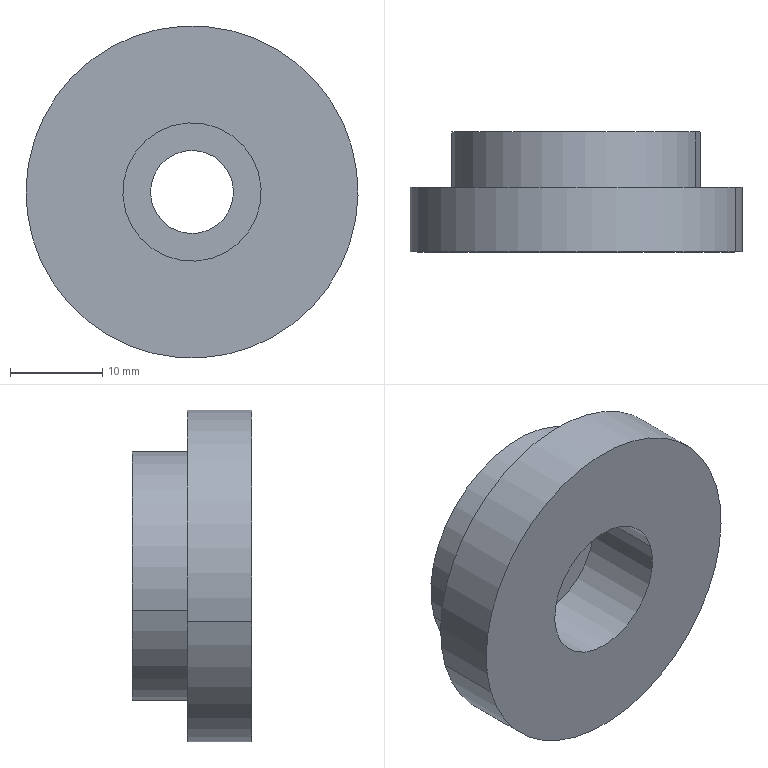Component | SolidWorks | NewDieSet-1_SpacerBlock-1 | 1 solid | 12 faces | box 36 x 13 x 36 mm | volume 8716 mm3 | cylinder 8 | plane 4 | commonest cylinder face diameters 15 x2 9 x2 27 x2 36 x2
build123d program:
from build123d import *

# Parameters (mm, degrees)
SKETCH1_R                                            = 18
BOSS_EXTRUDE1_DEPTH                                  = 7
SKETCH4_R                                            = 13.5
BOSS_EXTRUDE2_DEPTH                                  = 6
HOLE_SIZE_ACCORDING_TO_HEXAGON_SOCKET_HE_D           = 9
HOLE_SIZE_ACCORDING_TO_HEXAGON_SOCKET_HE_CBORE_D     = 15
HOLE_SIZE_ACCORDING_TO_HEXAGON_SOCKET_HE_CBORE_DEPTH = 9


with BuildPart() as part:
    # Sketch1 → Boss-Extrude1 (new body)
    with BuildSketch(Plane.XY):
        Circle(SKETCH1_R)
    extrude(amount=BOSS_EXTRUDE1_DEPTH)

    # Sketch4 → Boss-Extrude2 (add)
    with BuildSketch(Plane(origin=(0, 0, 0), x_dir=(-1, 0, 0), z_dir=(0, 0, -1))):
        with Locations(Location((0, 0, 0), (0, 0, 180))):
            Circle(SKETCH4_R)
    extrude(amount=BOSS_EXTRUDE2_DEPTH)

    # Hole Size_According to_Hexagon Socket He (through all)
    with Locations(Plane.XY.offset(7)):
        with Locations((0, 0)):
            CounterBoreHole(HOLE_SIZE_ACCORDING_TO_HEXAGON_SOCKET_HE_D / 2, HOLE_SIZE_ACCORDING_TO_HEXAGON_SOCKET_HE_CBORE_D / 2, HOLE_SIZE_ACCORDING_TO_HEXAGON_SOCKET_HE_CBORE_DEPTH)


solid = part.part

# Placed as in the assembly
solid = solid.moved(Location((68.254, -44.073, 138), (90, 0, 0)))
STEP:
#1=CARTESIAN_POINT('',(2.971,-1.656,5.515));
#2=VERTEX_POINT('',#1);
#3=CARTESIAN_POINT('',(2.403,-1.656,5.351));
#4=VERTEX_POINT('',#3);
#5=CARTESIAN_POINT('',(2.687,-1.656,5.433));
#6=DIRECTION('',(0.,-1.,0.));
#7=DIRECTION('',(-0.9609,0.,-0.2768));
#8=AXIS2_PLACEMENT_3D('',#5,#6,#7);
#9=CIRCLE('',#8,0.2953);
#10=EDGE_CURVE('',#2,#4,#9,.T.);
#11=ORIENTED_EDGE('',*,*,#10,.F.);
#12=CARTESIAN_POINT('',(2.971,-2.011,5.515));
#13=VERTEX_POINT('',#12);
#14=CARTESIAN_POINT('',(2.971,-2.011,5.515));
#15=DIRECTION('',(0.,-1.,0.));
#16=VECTOR('',#15,39.37);
#17=LINE('',#14,#16);
#18=EDGE_CURVE('',#2,#13,#17,.T.);
#19=ORIENTED_EDGE('',*,*,#18,.T.);
#20=CARTESIAN_POINT('',(2.403,-2.011,5.351));
#21=VERTEX_POINT('',#20);
#22=CARTESIAN_POINT('',(2.687,-2.011,5.433));
#23=DIRECTION('',(0.,-1.,0.));
#24=DIRECTION('',(-0.9609,0.,-0.2768));
#25=AXIS2_PLACEMENT_3D('',#22,#23,#24);
#26=CIRCLE('',#25,0.2953);
#27=EDGE_CURVE('',#13,#21,#26,.T.);
#28=ORIENTED_EDGE('',*,*,#27,.T.);
#29=CARTESIAN_POINT('',(2.403,-2.011,5.351));
#30=DIRECTION('',(0.,-1.,0.));
#31=VECTOR('',#30,39.37);
#32=LINE('',#29,#31);
#33=EDGE_CURVE('',#4,#21,#32,.T.);
#34=ORIENTED_EDGE('',*,*,#33,.F.);
#35=EDGE_LOOP('',(#11,#19,#28,#34));
#36=FACE_OUTER_BOUND('',#35,.T.);
#37=CARTESIAN_POINT('',(2.687,-2.011,5.433));
#38=DIRECTION('',(0.,-1.,0.));
#39=DIRECTION('',(-0.9609,0.,-0.2768));
#40=AXIS2_PLACEMENT_3D('',#37,#38,#39);
#41=CYLINDRICAL_SURFACE('',#40,0.2953);
#42=ADVANCED_FACE('',(#36),#41,.F.);
#43=CARTESIAN_POINT('',(2.857,-1.499,5.482));
#44=VERTEX_POINT('',#43);
#45=CARTESIAN_POINT('',(2.517,-1.499,5.384));
#46=VERTEX_POINT('',#45);
#47=CARTESIAN_POINT('',(2.687,-1.499,5.433));
#48=DIRECTION('',(0.,-1.,0.));
#49=DIRECTION('',(-0.9609,0.,-0.2768));
#50=AXIS2_PLACEMENT_3D('',#47,#48,#49);
#51=CIRCLE('',#50,0.1772);
#52=EDGE_CURVE('',#44,#46,#51,.T.);
#53=ORIENTED_EDGE('',*,*,#52,.F.);
#54=CARTESIAN_POINT('',(2.857,-1.656,5.482));
#55=VERTEX_POINT('',#54);
#56=CARTESIAN_POINT('',(2.857,-2.011,5.482));
#57=DIRECTION('',(0.,-1.,0.));
#58=VECTOR('',#57,39.37);
#59=LINE('',#56,#58);
#60=EDGE_CURVE('',#44,#55,#59,.T.);
#61=ORIENTED_EDGE('',*,*,#60,.T.);
#62=CARTESIAN_POINT('',(2.517,-1.656,5.384));
#63=VERTEX_POINT('',#62);
#64=CARTESIAN_POINT('',(2.687,-1.656,5.433));
#65=DIRECTION('',(0.,-1.,0.));
#66=DIRECTION('',(-0.9609,0.,-0.2768));
#67=AXIS2_PLACEMENT_3D('',#64,#65,#66);
#68=CIRCLE('',#67,0.1772);
#69=EDGE_CURVE('',#55,#63,#68,.T.);
#70=ORIENTED_EDGE('',*,*,#69,.T.);
#71=CARTESIAN_POINT('',(2.517,-2.011,5.384));
#72=DIRECTION('',(0.,-1.,0.));
#73=VECTOR('',#72,39.37);
#74=LINE('',#71,#73);
#75=EDGE_CURVE('',#46,#63,#74,.T.);
#76=ORIENTED_EDGE('',*,*,#75,.F.);
#77=EDGE_LOOP('',(#53,#61,#70,#76));
#78=FACE_OUTER_BOUND('',#77,.T.);
#79=CARTESIAN_POINT('',(2.687,-2.011,5.433));
#80=DIRECTION('',(0.,-1.,0.));
#81=DIRECTION('',(-0.9609,0.,-0.2768));
#82=AXIS2_PLACEMENT_3D('',#79,#80,#81);
#83=CYLINDRICAL_SURFACE('',#82,0.1772);
#84=ADVANCED_FACE('',(#78),#83,.F.);
#85=CARTESIAN_POINT('',(3.198,-1.499,5.58));
#86=VERTEX_POINT('',#85);
#87=CARTESIAN_POINT('',(2.176,-1.499,5.286));
#88=VERTEX_POINT('',#87);
#89=CARTESIAN_POINT('',(2.687,-1.499,5.433));
#90=DIRECTION('',(0.,1.,0.));
#91=DIRECTION('',(0.9609,0.,0.2768));
#92=AXIS2_PLACEMENT_3D('',#89,#90,#91);
#93=CIRCLE('',#92,0.5315);
#94=EDGE_CURVE('',#86,#88,#93,.T.);
#95=ORIENTED_EDGE('',*,*,#94,.F.);
#96=CARTESIAN_POINT('',(3.198,-1.735,5.58));
#97=VERTEX_POINT('',#96);
#98=CARTESIAN_POINT('',(3.198,-1.499,5.58));
#99=DIRECTION('',(0.,-1.,0.));
#100=VECTOR('',#99,39.37);
#101=LINE('',#98,#100);
#102=EDGE_CURVE('',#86,#97,#101,.T.);
#103=ORIENTED_EDGE('',*,*,#102,.T.);
#104=CARTESIAN_POINT('',(2.176,-1.735,5.286));
#105=VERTEX_POINT('',#104);
#106=CARTESIAN_POINT('',(2.687,-1.735,5.433));
#107=DIRECTION('',(0.,1.,0.));
#108=DIRECTION('',(-0.9609,0.,-0.2768));
#109=AXIS2_PLACEMENT_3D('',#106,#107,#108);
#110=CIRCLE('',#109,0.5315);
#111=EDGE_CURVE('',#97,#105,#110,.T.);
#112=ORIENTED_EDGE('',*,*,#111,.T.);
#113=CARTESIAN_POINT('',(2.176,-1.499,5.286));
#114=DIRECTION('',(0.,-1.,0.));
#115=VECTOR('',#114,39.37);
#116=LINE('',#113,#115);
#117=EDGE_CURVE('',#88,#105,#116,.T.);
#118=ORIENTED_EDGE('',*,*,#117,.F.);
#119=EDGE_LOOP('',(#95,#103,#112,#118));
#120=FACE_OUTER_BOUND('',#119,.T.);
#121=CARTESIAN_POINT('',(2.687,-1.499,5.433));
#122=DIRECTION('',(0.,-1.,0.));
#123=DIRECTION('',(-0.9609,0.,-0.2768));
#124=AXIS2_PLACEMENT_3D('',#121,#122,#123);
#125=CYLINDRICAL_SURFACE('',#124,0.5315);
#126=ADVANCED_FACE('',(#120),#125,.T.);
#127=CARTESIAN_POINT('',(2.006,-2.011,5.237));
#128=VERTEX_POINT('',#127);
#129=CARTESIAN_POINT('',(3.368,-2.011,5.629));
#130=VERTEX_POINT('',#129);
#131=CARTESIAN_POINT('',(2.687,-2.011,5.433));
#132=DIRECTION('',(0.,-1.,0.));
#133=DIRECTION('',(-0.9609,0.,-0.2768));
#134=AXIS2_PLACEMENT_3D('',#131,#132,#133);
#135=CIRCLE('',#134,0.7087);
#136=EDGE_CURVE('',#128,#130,#135,.T.);
#137=ORIENTED_EDGE('',*,*,#136,.F.);
#138=CARTESIAN_POINT('',(2.006,-1.735,5.237));
#139=VERTEX_POINT('',#138);
#140=CARTESIAN_POINT('',(2.006,-2.011,5.237));
#141=DIRECTION('',(0.,1.,0.));
#142=VECTOR('',#141,39.37);
#143=LINE('',#140,#142);
#144=EDGE_CURVE('',#128,#139,#143,.T.);
#145=ORIENTED_EDGE('',*,*,#144,.T.);
#146=CARTESIAN_POINT('',(3.368,-1.735,5.629));
#147=VERTEX_POINT('',#146);
#148=CARTESIAN_POINT('',(2.687,-1.735,5.433));
#149=DIRECTION('',(0.,-1.,0.));
#150=DIRECTION('',(-0.9609,0.,-0.2768));
#151=AXIS2_PLACEMENT_3D('',#148,#149,#150);
#152=CIRCLE('',#151,0.7087);
#153=EDGE_CURVE('',#139,#147,#152,.T.);
#154=ORIENTED_EDGE('',*,*,#153,.T.);
#155=CARTESIAN_POINT('',(3.368,-2.011,5.629));
#156=DIRECTION('',(0.,1.,0.));
#157=VECTOR('',#156,39.37);
#158=LINE('',#155,#157);
#159=EDGE_CURVE('',#130,#147,#158,.T.);
#160=ORIENTED_EDGE('',*,*,#159,.F.);
#161=EDGE_LOOP('',(#137,#145,#154,#160));
#162=FACE_OUTER_BOUND('',#161,.T.);
#163=CARTESIAN_POINT('',(2.687,-2.011,5.433));
#164=DIRECTION('',(0.,1.,0.));
#165=DIRECTION('',(0.9609,0.,0.2768));
#166=AXIS2_PLACEMENT_3D('',#163,#164,#165);
#167=CYLINDRICAL_SURFACE('',#166,0.7087);
#168=ADVANCED_FACE('',(#162),#167,.T.);
#169=ORIENTED_EDGE('',*,*,#144,.F.);
#170=CARTESIAN_POINT('',(2.687,-2.011,5.433));
#171=DIRECTION('',(0.,-1.,0.));
#172=DIRECTION('',(-0.9609,0.,-0.2768));
#173=AXIS2_PLACEMENT_3D('',#170,#171,#172);
#174=CIRCLE('',#173,0.7087);
#175=EDGE_CURVE('',#130,#128,#174,.T.);
#176=ORIENTED_EDGE('',*,*,#175,.F.);
#177=ORIENTED_EDGE('',*,*,#159,.T.);
#178=CARTESIAN_POINT('',(2.687,-1.735,5.433));
#179=DIRECTION('',(0.,-1.,0.));
#180=DIRECTION('',(-0.9609,0.,-0.2768));
#181=AXIS2_PLACEMENT_3D('',#178,#179,#180);
#182=CIRCLE('',#181,0.7087);
#183=EDGE_CURVE('',#147,#139,#182,.T.);
#184=ORIENTED_EDGE('',*,*,#183,.T.);
#185=EDGE_LOOP('',(#169,#176,#177,#184));
#186=FACE_OUTER_BOUND('',#185,.T.);
#187=CARTESIAN_POINT('',(2.687,-2.011,5.433));
#188=DIRECTION('',(0.,1.,0.));
#189=DIRECTION('',(0.9609,0.,0.2768));
#190=AXIS2_PLACEMENT_3D('',#187,#188,#189);
#191=CYLINDRICAL_SURFACE('',#190,0.7087);
#192=ADVANCED_FACE('',(#186),#191,.T.);
#193=CARTESIAN_POINT('',(2.687,-2.011,5.433));
#194=DIRECTION('',(0.,-1.,0.));
#195=DIRECTION('',(-0.9609,0.,-0.2768));
#196=AXIS2_PLACEMENT_3D('',#193,#194,#195);
#197=CIRCLE('',#196,0.2953);
#198=EDGE_CURVE('',#21,#13,#197,.T.);
#199=ORIENTED_EDGE('',*,*,#198,.F.);
#200=ORIENTED_EDGE('',*,*,#27,.F.);
#201=EDGE_LOOP('',(#199,#200));
#202=FACE_BOUND('',#201,.T.);
#203=ORIENTED_EDGE('',*,*,#175,.T.);
#204=ORIENTED_EDGE('',*,*,#136,.T.);
#205=EDGE_LOOP('',(#203,#204));
#206=FACE_OUTER_BOUND('',#205,.T.);
#207=CARTESIAN_POINT('',(2.687,-2.011,5.433));
#208=DIRECTION('',(0.,-1.,0.));
#209=DIRECTION('',(-0.9609,0.,-0.2768));
#210=AXIS2_PLACEMENT_3D('',#207,#208,#209);
#211=PLANE('',#210);
#212=ADVANCED_FACE('',(#202,#206),#211,.T.);
#213=CARTESIAN_POINT('',(2.687,-1.735,5.433));
#214=DIRECTION('',(0.,1.,0.));
#215=DIRECTION('',(-0.9609,0.,-0.2768));
#216=AXIS2_PLACEMENT_3D('',#213,#214,#215);
#217=CIRCLE('',#216,0.5315);
#218=EDGE_CURVE('',#105,#97,#217,.T.);
#219=ORIENTED_EDGE('',*,*,#218,.F.);
#220=ORIENTED_EDGE('',*,*,#111,.F.);
#221=EDGE_LOOP('',(#219,#220));
#222=FACE_BOUND('',#221,.T.);
#223=ORIENTED_EDGE('',*,*,#183,.F.);
#224=ORIENTED_EDGE('',*,*,#153,.F.);
#225=EDGE_LOOP('',(#223,#224));
#226=FACE_OUTER_BOUND('',#225,.T.);
#227=CARTESIAN_POINT('',(2.687,-1.735,5.433));
#228=DIRECTION('',(0.,-1.,0.));
#229=DIRECTION('',(-0.9609,0.,-0.2768));
#230=AXIS2_PLACEMENT_3D('',#227,#228,#229);
#231=PLANE('',#230);
#232=ADVANCED_FACE('',(#222,#226),#231,.F.);
#233=ORIENTED_EDGE('',*,*,#102,.F.);
#234=CARTESIAN_POINT('',(2.687,-1.499,5.433));
#235=DIRECTION('',(0.,1.,0.));
#236=DIRECTION('',(0.9609,0.,0.2768));
#237=AXIS2_PLACEMENT_3D('',#234,#235,#236);
#238=CIRCLE('',#237,0.5315);
#239=EDGE_CURVE('',#88,#86,#238,.T.);
#240=ORIENTED_EDGE('',*,*,#239,.F.);
#241=ORIENTED_EDGE('',*,*,#117,.T.);
#242=ORIENTED_EDGE('',*,*,#218,.T.);
#243=EDGE_LOOP('',(#233,#240,#241,#242));
#244=FACE_OUTER_BOUND('',#243,.T.);
#245=CARTESIAN_POINT('',(2.687,-1.499,5.433));
#246=DIRECTION('',(0.,-1.,0.));
#247=DIRECTION('',(-0.9609,0.,-0.2768));
#248=AXIS2_PLACEMENT_3D('',#245,#246,#247);
#249=CYLINDRICAL_SURFACE('',#248,0.5315);
#250=ADVANCED_FACE('',(#244),#249,.T.);
#251=CARTESIAN_POINT('',(2.687,-1.499,5.433));
#252=DIRECTION('',(0.,-1.,0.));
#253=DIRECTION('',(-0.9609,0.,-0.2768));
#254=AXIS2_PLACEMENT_3D('',#251,#252,#253);
#255=CIRCLE('',#254,0.1772);
#256=EDGE_CURVE('',#46,#44,#255,.T.);
#257=ORIENTED_EDGE('',*,*,#256,.T.);
#258=ORIENTED_EDGE('',*,*,#52,.T.);
#259=EDGE_LOOP('',(#257,#258));
#260=FACE_BOUND('',#259,.T.);
#261=ORIENTED_EDGE('',*,*,#239,.T.);
#262=ORIENTED_EDGE('',*,*,#94,.T.);
#263=EDGE_LOOP('',(#261,#262));
#264=FACE_OUTER_BOUND('',#263,.T.);
#265=CARTESIAN_POINT('',(2.687,-1.499,5.433));
#266=DIRECTION('',(0.,1.,0.));
#267=DIRECTION('',(0.9609,0.,0.2768));
#268=AXIS2_PLACEMENT_3D('',#265,#266,#267);
#269=PLANE('',#268);
#270=ADVANCED_FACE('',(#260,#264),#269,.T.);
#271=ORIENTED_EDGE('',*,*,#60,.F.);
#272=ORIENTED_EDGE('',*,*,#256,.F.);
#273=ORIENTED_EDGE('',*,*,#75,.T.);
#274=CARTESIAN_POINT('',(2.687,-1.656,5.433));
#275=DIRECTION('',(0.,-1.,0.));
#276=DIRECTION('',(-0.9609,0.,-0.2768));
#277=AXIS2_PLACEMENT_3D('',#274,#275,#276);
#278=CIRCLE('',#277,0.1772);
#279=EDGE_CURVE('',#63,#55,#278,.T.);
#280=ORIENTED_EDGE('',*,*,#279,.T.);
#281=EDGE_LOOP('',(#271,#272,#273,#280));
#282=FACE_OUTER_BOUND('',#281,.T.);
#283=CARTESIAN_POINT('',(2.687,-2.011,5.433));
#284=DIRECTION('',(0.,-1.,0.));
#285=DIRECTION('',(-0.9609,0.,-0.2768));
#286=AXIS2_PLACEMENT_3D('',#283,#284,#285);
#287=CYLINDRICAL_SURFACE('',#286,0.1772);
#288=ADVANCED_FACE('',(#282),#287,.F.);
#289=ORIENTED_EDGE('',*,*,#279,.F.);
#290=ORIENTED_EDGE('',*,*,#69,.F.);
#291=EDGE_LOOP('',(#289,#290));
#292=FACE_BOUND('',#291,.T.);
#293=CARTESIAN_POINT('',(2.687,-1.656,5.433));
#294=DIRECTION('',(0.,-1.,0.));
#295=DIRECTION('',(-0.9609,0.,-0.2768));
#296=AXIS2_PLACEMENT_3D('',#293,#294,#295);
#297=CIRCLE('',#296,0.2953);
#298=EDGE_CURVE('',#4,#2,#297,.T.);
#299=ORIENTED_EDGE('',*,*,#298,.T.);
#300=ORIENTED_EDGE('',*,*,#10,.T.);
#301=EDGE_LOOP('',(#299,#300));
#302=FACE_OUTER_BOUND('',#301,.T.);
#303=CARTESIAN_POINT('',(2.517,-1.656,5.384));
#304=DIRECTION('',(0.,1.,0.));
#305=DIRECTION('',(0.9609,0.,0.2768));
#306=AXIS2_PLACEMENT_3D('',#303,#304,#305);
#307=PLANE('',#306);
#308=ADVANCED_FACE('',(#292,#302),#307,.F.);
#309=ORIENTED_EDGE('',*,*,#18,.F.);
#310=ORIENTED_EDGE('',*,*,#298,.F.);
#311=ORIENTED_EDGE('',*,*,#33,.T.);
#312=ORIENTED_EDGE('',*,*,#198,.T.);
#313=EDGE_LOOP('',(#309,#310,#311,#312));
#314=FACE_OUTER_BOUND('',#313,.T.);
#315=CARTESIAN_POINT('',(2.687,-2.011,5.433));
#316=DIRECTION('',(0.,-1.,0.));
#317=DIRECTION('',(-0.9609,0.,-0.2768));
#318=AXIS2_PLACEMENT_3D('',#315,#316,#317);
#319=CYLINDRICAL_SURFACE('',#318,0.2953);
#320=ADVANCED_FACE('',(#314),#319,.F.);
#321=CLOSED_SHELL('',(#42,#84,#126,#168,#192,#212,#232,#250,#270,#288,#308,#320));
#322=MANIFOLD_SOLID_BREP('',#321);
#323=CARTESIAN_POINT('',(0.,0.,0.));
#324=DIRECTION('',(0.,0.,1.));
#325=DIRECTION('',(1.,0.,0.));
#326=AXIS2_PLACEMENT_3D('',#323,#324,#325);
#327=(LENGTH_UNIT()NAMED_UNIT(*)SI_UNIT($,.METRE.));
#328=LENGTH_MEASURE_WITH_UNIT(LENGTH_MEASURE(0.0254),#327);
#329=DIMENSIONAL_EXPONENTS(1.,0.,0.,0.,0.,0.,0.);
#330=(CONVERSION_BASED_UNIT('',#328)LENGTH_UNIT()NAMED_UNIT(#329));
#331=UNCERTAINTY_MEASURE_WITH_UNIT(LENGTH_MEASURE(0.00001),#330,'','');
#332=(NAMED_UNIT(*)PLANE_ANGLE_UNIT()SI_UNIT($,.RADIAN.));
#333=(NAMED_UNIT(*)SI_UNIT($,.STERADIAN.)SOLID_ANGLE_UNIT());
#334=(GEOMETRIC_REPRESENTATION_CONTEXT(3)GLOBAL_UNCERTAINTY_ASSIGNED_CONTEXT((#331))GLOBAL_UNIT_ASSIGNED_CONTEXT((#330,#332,#333))REPRESENTATION_CONTEXT('',''));
#335=ADVANCED_BREP_SHAPE_REPRESENTATION('',(#322,#326),#334);
#336=COLOUR_RGB('',0.7922,0.8196,0.9333);
#337=FILL_AREA_STYLE_COLOUR('',#336);
#338=FILL_AREA_STYLE('',(#337));
#339=SURFACE_STYLE_FILL_AREA(#338);
#340=SURFACE_SIDE_STYLE('',(#339));
#341=SURFACE_STYLE_USAGE(.BOTH.,#340);
#342=PRESENTATION_STYLE_ASSIGNMENT((#341));
#343=STYLED_ITEM('',(#342),#322);
#344=PRESENTATION_LAYER_ASSIGNMENT('','',(#343));
#345=(LENGTH_UNIT()NAMED_UNIT(*)SI_UNIT($,.METRE.));
#346=LENGTH_MEASURE_WITH_UNIT(LENGTH_MEASURE(0.0254),#345);
#347=DIMENSIONAL_EXPONENTS(1.,0.,0.,0.,0.,0.,0.);
#348=(CONVERSION_BASED_UNIT('',#346)LENGTH_UNIT()NAMED_UNIT(#347));
#349=UNCERTAINTY_MEASURE_WITH_UNIT(LENGTH_MEASURE(0.00001),#348,'','');
#350=(NAMED_UNIT(*)PLANE_ANGLE_UNIT()SI_UNIT($,.RADIAN.));
#351=(NAMED_UNIT(*)SI_UNIT($,.STERADIAN.)SOLID_ANGLE_UNIT());
#352=(GEOMETRIC_REPRESENTATION_CONTEXT(3)GLOBAL_UNCERTAINTY_ASSIGNED_CONTEXT((#349))GLOBAL_UNIT_ASSIGNED_CONTEXT((#348,#350,#351))REPRESENTATION_CONTEXT('',''));
#353=MECHANICAL_DESIGN_GEOMETRIC_PRESENTATION_REPRESENTATION('',(#343),#352);